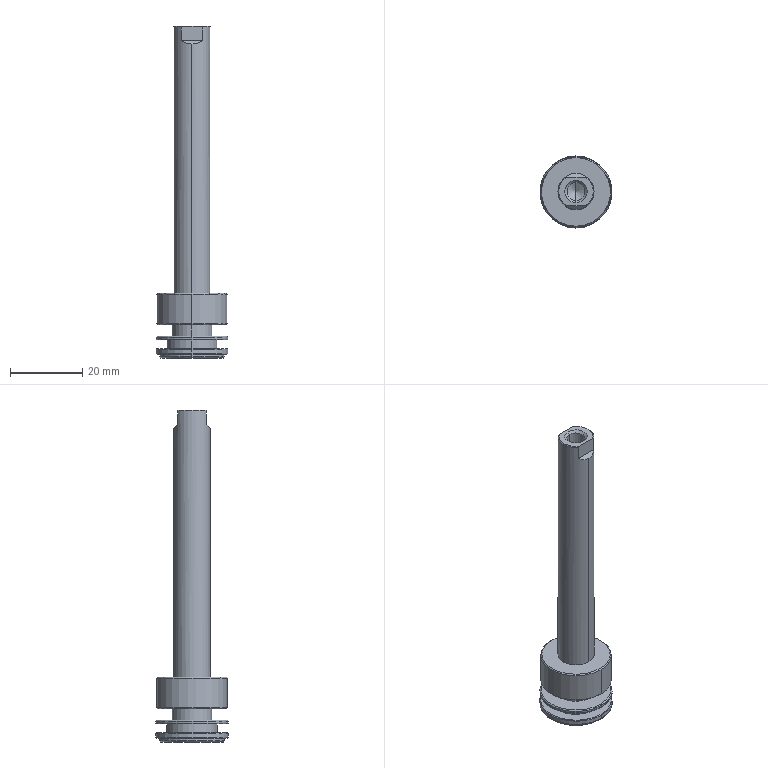Component | SolidWorks | ACQS_20x60_0-2_ACQS_20x60_60r-1 | 1 solid | 48 faces | volume 9991 mm3 | cylinder 16 | cone 12 | plane 12 | torus 8 | commonest cylinder face diameters 20 x4 5 x2 18 x2 14 x2 11 x2 19.6 x2 10 x2